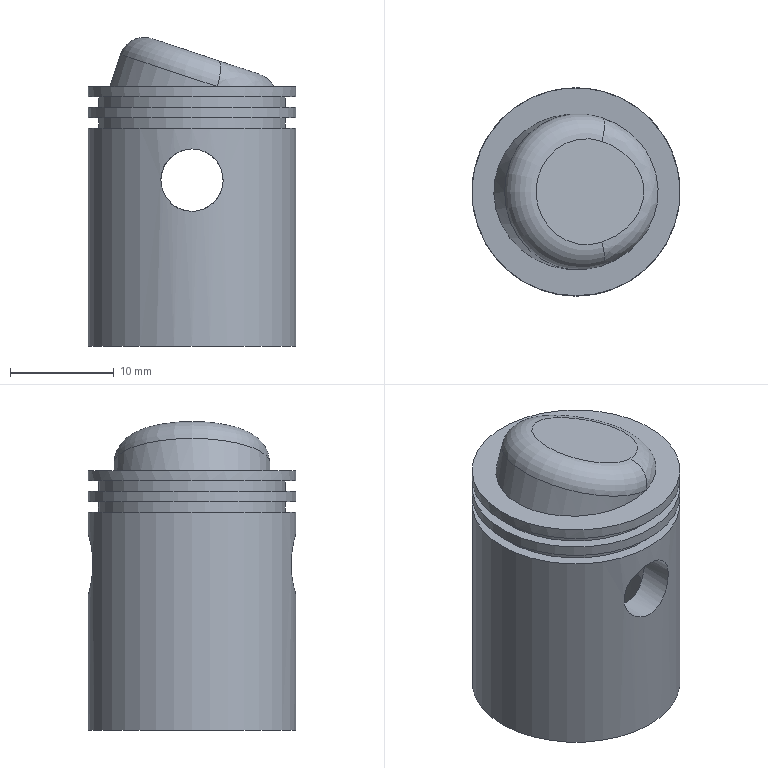Component | NX | PISTON | 1 solid | 21 faces | volume 3115 mm3 | cylinder 10 | plane 8 | cone 1 | torus 1 | spline 1 | commonest cylinder face diameters 20 x3 18 x3 6 x2 14 x1 15 x1